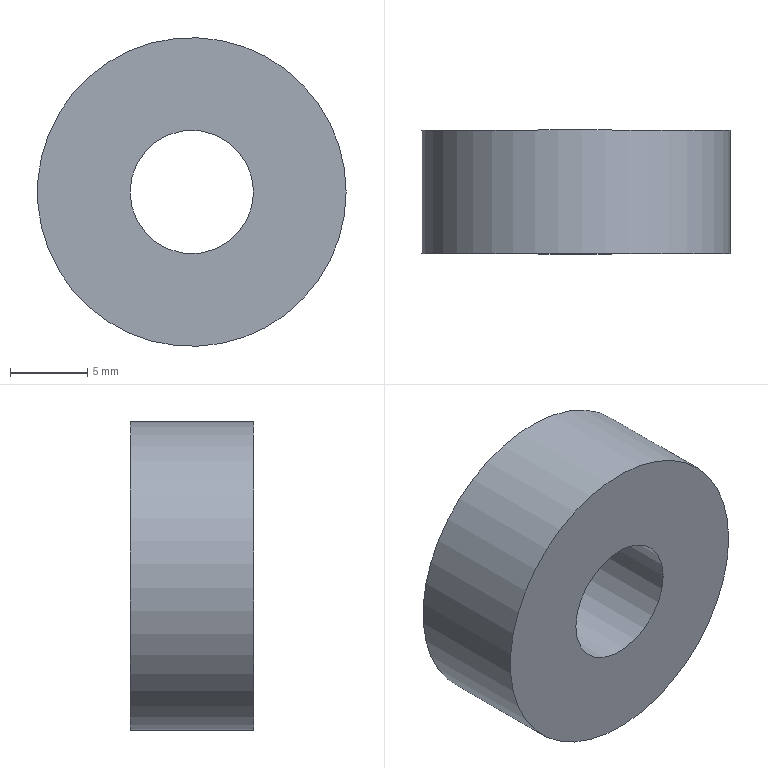Component | NX | IDLER_WHEEL | 1 solid | 4 faces | box 20 x 8 x 20 mm | volume 2111 mm3 | cylinder 2 | plane 2 | commonest cylinder face diameters 20 x1 8 x1
STEP:
#1=CARTESIAN_POINT('',(0.,0.,0.));
#2=DIRECTION('',(0.,0.,1.));
#3=DIRECTION('',(1.,0.,0.));
#4=AXIS2_PLACEMENT_3D('',#1,#2,#3);
#5=CARTESIAN_POINT('',(-63.,-4.,-1.));
#6=VERTEX_POINT('',#5);
#7=CARTESIAN_POINT('',(-73.,-4.,-1.));
#8=DIRECTION('',(0.,-1.,0.));
#9=DIRECTION('',(1.,0.,0.));
#10=AXIS2_PLACEMENT_3D('',#7,#8,#9);
#11=CIRCLE('',#10,10.);
#12=CARTESIAN_POINT('',(-73.,-4.,-1.));
#13=DIRECTION('',(0.,1.,0.));
#14=DIRECTION('',(-1.,0.,0.));
#15=AXIS2_PLACEMENT_3D('',#12,#13,#14);
#16=CYLINDRICAL_SURFACE('',#15,10.);
#17=CARTESIAN_POINT('',(9.425,0.));
#18=DIRECTION('',(-1.,0.));
#19=VECTOR('',#18,1.);
#20=LINE('',#17,#19);
#21=(GEOMETRIC_REPRESENTATION_CONTEXT(2)PARAMETRIC_REPRESENTATION_CONTEXT()REPRESENTATION_CONTEXT('',''));
#22=DEFINITIONAL_REPRESENTATION('',(#20),#21);
#23=PCURVE('',#16,#22);
#24=CARTESIAN_POINT('',(-73.,-4.,-1.));
#25=DIRECTION('',(0.,-1.,0.));
#26=DIRECTION('',(1.,0.,0.));
#27=AXIS2_PLACEMENT_3D('',#24,#25,#26);
#28=PLANE('',#27);
#29=CARTESIAN_POINT('',(0.,0.));
#30=DIRECTION('',(1.,0.));
#31=AXIS2_PLACEMENT_2D('',#29,#30);
#32=CIRCLE('',#31,10.);
#33=(GEOMETRIC_REPRESENTATION_CONTEXT(2)PARAMETRIC_REPRESENTATION_CONTEXT()REPRESENTATION_CONTEXT('',''));
#34=DEFINITIONAL_REPRESENTATION('',(#32),#33);
#35=PCURVE('',#28,#34);
#36=SURFACE_CURVE('',#11,(#23,#35),.PCURVE_S1.);
#37=EDGE_CURVE('',#6,#6,#36,.T.);
#38=ORIENTED_EDGE('',*,*,#37,.F.);
#39=CARTESIAN_POINT('',(-63.,4.,-1.));
#40=VERTEX_POINT('',#39);
#41=CARTESIAN_POINT('',(-63.,-4.,-1.));
#42=CARTESIAN_POINT('',(-63.,4.,-1.));
#43=B_SPLINE_CURVE_WITH_KNOTS('',1,(#41,#42),.UNSPECIFIED.,.F.,.F.,(2,2),(0.,8.),.PIECEWISE_BEZIER_KNOTS.);
#44=CARTESIAN_POINT('',(9.425,0.));
#45=DIRECTION('',(0.,1.));
#46=VECTOR('',#45,1.);
#47=LINE('',#44,#46);
#48=(GEOMETRIC_REPRESENTATION_CONTEXT(2)PARAMETRIC_REPRESENTATION_CONTEXT()REPRESENTATION_CONTEXT('',''));
#49=DEFINITIONAL_REPRESENTATION('',(#47),#48);
#50=PCURVE('',#16,#49);
#51=CARTESIAN_POINT('',(3.142,0.));
#52=DIRECTION('',(0.,1.));
#53=VECTOR('',#52,1.);
#54=LINE('',#51,#53);
#55=(GEOMETRIC_REPRESENTATION_CONTEXT(2)PARAMETRIC_REPRESENTATION_CONTEXT()REPRESENTATION_CONTEXT('',''));
#56=DEFINITIONAL_REPRESENTATION('',(#54),#55);
#57=PCURVE('',#16,#56);
#58=SEAM_CURVE('',#43,(#50,#57),.PCURVE_S1.);
#59=EDGE_CURVE('',#6,#40,#58,.T.);
#60=ORIENTED_EDGE('',*,*,#59,.T.);
#61=CARTESIAN_POINT('',(-73.,4.,-1.));
#62=DIRECTION('',(0.,-1.,0.));
#63=DIRECTION('',(1.,0.,0.));
#64=AXIS2_PLACEMENT_3D('',#61,#62,#63);
#65=CIRCLE('',#64,10.);
#66=CARTESIAN_POINT('',(9.425,8.));
#67=DIRECTION('',(-1.,0.));
#68=VECTOR('',#67,1.);
#69=LINE('',#66,#68);
#70=(GEOMETRIC_REPRESENTATION_CONTEXT(2)PARAMETRIC_REPRESENTATION_CONTEXT()REPRESENTATION_CONTEXT('',''));
#71=DEFINITIONAL_REPRESENTATION('',(#69),#70);
#72=PCURVE('',#16,#71);
#73=CARTESIAN_POINT('',(-73.,4.,-1.));
#74=DIRECTION('',(0.,-1.,0.));
#75=DIRECTION('',(1.,0.,0.));
#76=AXIS2_PLACEMENT_3D('',#73,#74,#75);
#77=PLANE('',#76);
#78=CARTESIAN_POINT('',(0.,0.));
#79=DIRECTION('',(1.,0.));
#80=AXIS2_PLACEMENT_2D('',#78,#79);
#81=CIRCLE('',#80,10.);
#82=(GEOMETRIC_REPRESENTATION_CONTEXT(2)PARAMETRIC_REPRESENTATION_CONTEXT()REPRESENTATION_CONTEXT('',''));
#83=DEFINITIONAL_REPRESENTATION('',(#81),#82);
#84=PCURVE('',#77,#83);
#85=SURFACE_CURVE('',#65,(#72,#84),.PCURVE_S1.);
#86=EDGE_CURVE('',#40,#40,#85,.T.);
#87=ORIENTED_EDGE('',*,*,#86,.T.);
#88=ORIENTED_EDGE('',*,*,#59,.F.);
#89=EDGE_LOOP('',(#38,#60,#87,#88));
#90=FACE_BOUND('',#89,.T.);
#91=ADVANCED_FACE('',(#90),#16,.T.);
#92=CARTESIAN_POINT('',(-69.,-4.,-1.));
#93=VERTEX_POINT('',#92);
#94=CARTESIAN_POINT('',(-73.,-4.,-1.));
#95=DIRECTION('',(0.,-1.,0.));
#96=DIRECTION('',(1.,0.,0.));
#97=AXIS2_PLACEMENT_3D('',#94,#95,#96);
#98=CIRCLE('',#97,4.);
#99=CARTESIAN_POINT('',(-73.,-4.,-1.));
#100=DIRECTION('',(0.,1.,0.));
#101=DIRECTION('',(-1.,0.,0.));
#102=AXIS2_PLACEMENT_3D('',#99,#100,#101);
#103=CYLINDRICAL_SURFACE('',#102,4.);
#104=CARTESIAN_POINT('',(9.425,0.));
#105=DIRECTION('',(-1.,0.));
#106=VECTOR('',#105,1.);
#107=LINE('',#104,#106);
#108=(GEOMETRIC_REPRESENTATION_CONTEXT(2)PARAMETRIC_REPRESENTATION_CONTEXT()REPRESENTATION_CONTEXT('',''));
#109=DEFINITIONAL_REPRESENTATION('',(#107),#108);
#110=PCURVE('',#103,#109);
#111=CARTESIAN_POINT('',(0.,0.));
#112=DIRECTION('',(1.,0.));
#113=AXIS2_PLACEMENT_2D('',#111,#112);
#114=CIRCLE('',#113,4.);
#115=(GEOMETRIC_REPRESENTATION_CONTEXT(2)PARAMETRIC_REPRESENTATION_CONTEXT()REPRESENTATION_CONTEXT('',''));
#116=DEFINITIONAL_REPRESENTATION('',(#114),#115);
#117=PCURVE('',#28,#116);
#118=SURFACE_CURVE('',#98,(#110,#117),.PCURVE_S1.);
#119=EDGE_CURVE('',#93,#93,#118,.T.);
#120=ORIENTED_EDGE('',*,*,#119,.F.);
#121=CARTESIAN_POINT('',(-69.,4.,-1.));
#122=VERTEX_POINT('',#121);
#123=CARTESIAN_POINT('',(-69.,-4.,-1.));
#124=CARTESIAN_POINT('',(-69.,4.,-1.));
#125=B_SPLINE_CURVE_WITH_KNOTS('',1,(#123,#124),.UNSPECIFIED.,.F.,.F.,(2,2),(0.,8.),.PIECEWISE_BEZIER_KNOTS.);
#126=CARTESIAN_POINT('',(9.425,0.));
#127=DIRECTION('',(0.,1.));
#128=VECTOR('',#127,1.);
#129=LINE('',#126,#128);
#130=(GEOMETRIC_REPRESENTATION_CONTEXT(2)PARAMETRIC_REPRESENTATION_CONTEXT()REPRESENTATION_CONTEXT('',''));
#131=DEFINITIONAL_REPRESENTATION('',(#129),#130);
#132=PCURVE('',#103,#131);
#133=CARTESIAN_POINT('',(3.142,0.));
#134=DIRECTION('',(0.,1.));
#135=VECTOR('',#134,1.);
#136=LINE('',#133,#135);
#137=(GEOMETRIC_REPRESENTATION_CONTEXT(2)PARAMETRIC_REPRESENTATION_CONTEXT()REPRESENTATION_CONTEXT('',''));
#138=DEFINITIONAL_REPRESENTATION('',(#136),#137);
#139=PCURVE('',#103,#138);
#140=SEAM_CURVE('',#125,(#132,#139),.PCURVE_S1.);
#141=EDGE_CURVE('',#93,#122,#140,.T.);
#142=ORIENTED_EDGE('',*,*,#141,.T.);
#143=CARTESIAN_POINT('',(-73.,4.,-1.));
#144=DIRECTION('',(0.,-1.,0.));
#145=DIRECTION('',(1.,0.,0.));
#146=AXIS2_PLACEMENT_3D('',#143,#144,#145);
#147=CIRCLE('',#146,4.);
#148=CARTESIAN_POINT('',(9.425,8.));
#149=DIRECTION('',(-1.,0.));
#150=VECTOR('',#149,1.);
#151=LINE('',#148,#150);
#152=(GEOMETRIC_REPRESENTATION_CONTEXT(2)PARAMETRIC_REPRESENTATION_CONTEXT()REPRESENTATION_CONTEXT('',''));
#153=DEFINITIONAL_REPRESENTATION('',(#151),#152);
#154=PCURVE('',#103,#153);
#155=CARTESIAN_POINT('',(0.,0.));
#156=DIRECTION('',(1.,0.));
#157=AXIS2_PLACEMENT_2D('',#155,#156);
#158=CIRCLE('',#157,4.);
#159=(GEOMETRIC_REPRESENTATION_CONTEXT(2)PARAMETRIC_REPRESENTATION_CONTEXT()REPRESENTATION_CONTEXT('',''));
#160=DEFINITIONAL_REPRESENTATION('',(#158),#159);
#161=PCURVE('',#77,#160);
#162=SURFACE_CURVE('',#147,(#154,#161),.PCURVE_S1.);
#163=EDGE_CURVE('',#122,#122,#162,.T.);
#164=ORIENTED_EDGE('',*,*,#163,.T.);
#165=ORIENTED_EDGE('',*,*,#141,.F.);
#166=EDGE_LOOP('',(#120,#142,#164,#165));
#167=FACE_BOUND('',#166,.F.);
#168=ADVANCED_FACE('',(#167),#103,.F.);
#169=ORIENTED_EDGE('',*,*,#37,.T.);
#170=EDGE_LOOP('',(#169));
#171=FACE_BOUND('',#170,.T.);
#172=ORIENTED_EDGE('',*,*,#119,.F.);
#173=EDGE_LOOP('',(#172));
#174=FACE_BOUND('',#173,.T.);
#175=ADVANCED_FACE('',(#171,#174),#28,.T.);
#176=ORIENTED_EDGE('',*,*,#86,.F.);
#177=EDGE_LOOP('',(#176));
#178=FACE_BOUND('',#177,.T.);
#179=ORIENTED_EDGE('',*,*,#163,.T.);
#180=EDGE_LOOP('',(#179));
#181=FACE_BOUND('',#180,.T.);
#182=ADVANCED_FACE('',(#178,#181),#77,.F.);
#183=CLOSED_SHELL('',(#91,#168,#175,#182));
#184=MANIFOLD_SOLID_BREP('',#183);
#185=(LENGTH_UNIT()NAMED_UNIT(*)SI_UNIT(.MILLI.,.METRE.));
#186=UNCERTAINTY_MEASURE_WITH_UNIT(LENGTH_MEASURE(0.00001),#185,'','');
#187=(NAMED_UNIT(*)PLANE_ANGLE_UNIT()SI_UNIT($,.RADIAN.));
#188=(NAMED_UNIT(*)SI_UNIT($,.STERADIAN.)SOLID_ANGLE_UNIT());
#189=(GEOMETRIC_REPRESENTATION_CONTEXT(3)GLOBAL_UNCERTAINTY_ASSIGNED_CONTEXT((#186))GLOBAL_UNIT_ASSIGNED_CONTEXT((#185,#187,#188))REPRESENTATION_CONTEXT('',''));
#190=ADVANCED_BREP_SHAPE_REPRESENTATION('',(#4,#184),#189);